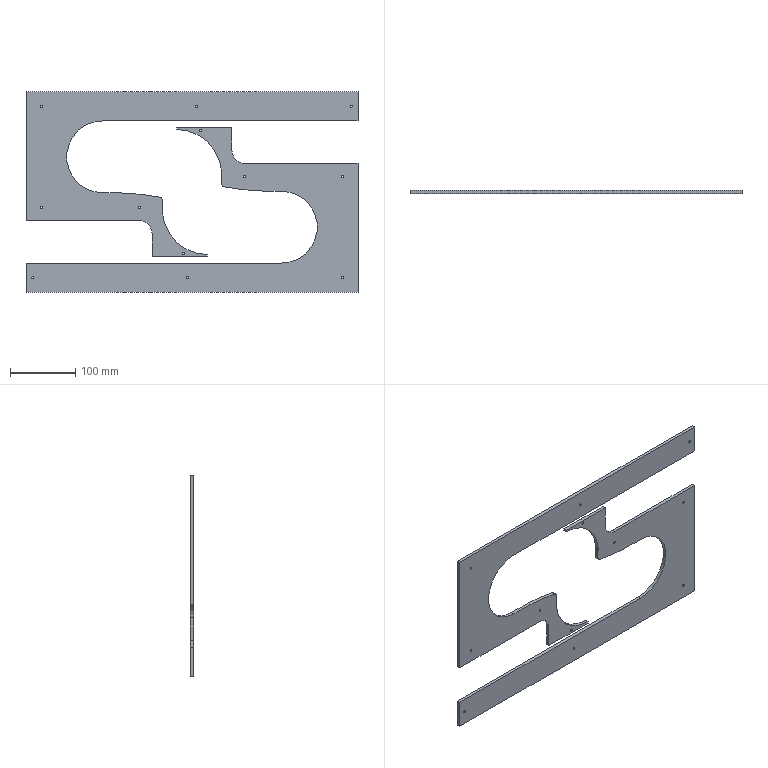CAM job | Mastercam | mm | 4 operations | part box 509.5 x 5 x 308
1. Contour (Ramp) | 3 - 3 平铣刀
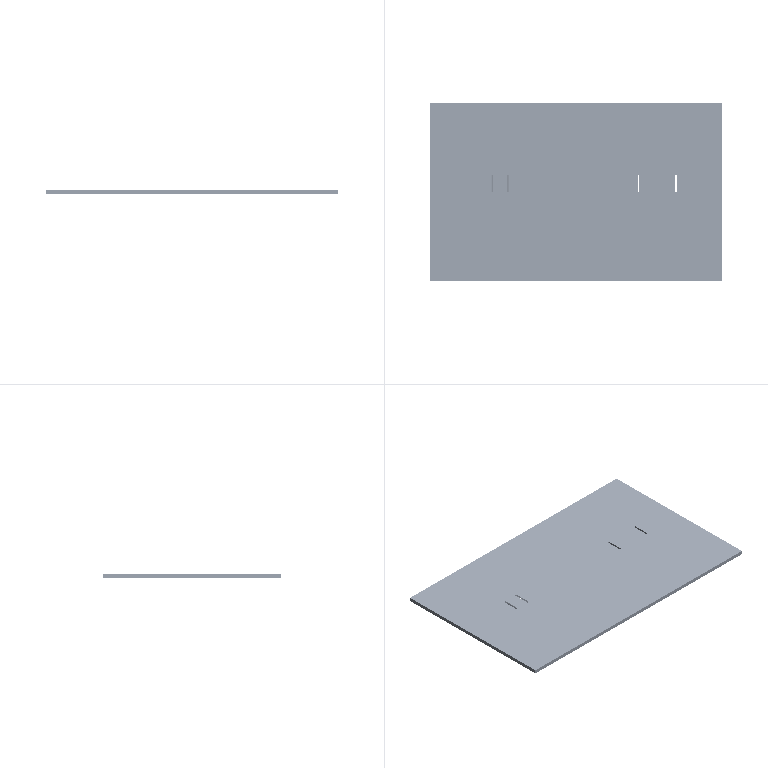2. Contour (2D) | 3 - 3 平铣刀
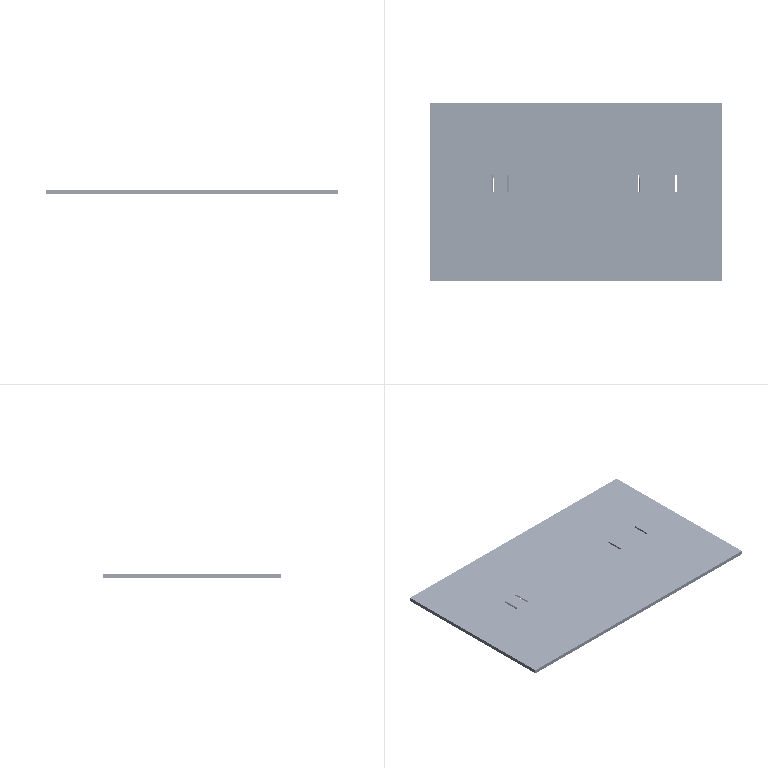3. Drill/Counterbore | 7 - 4 倒角刀
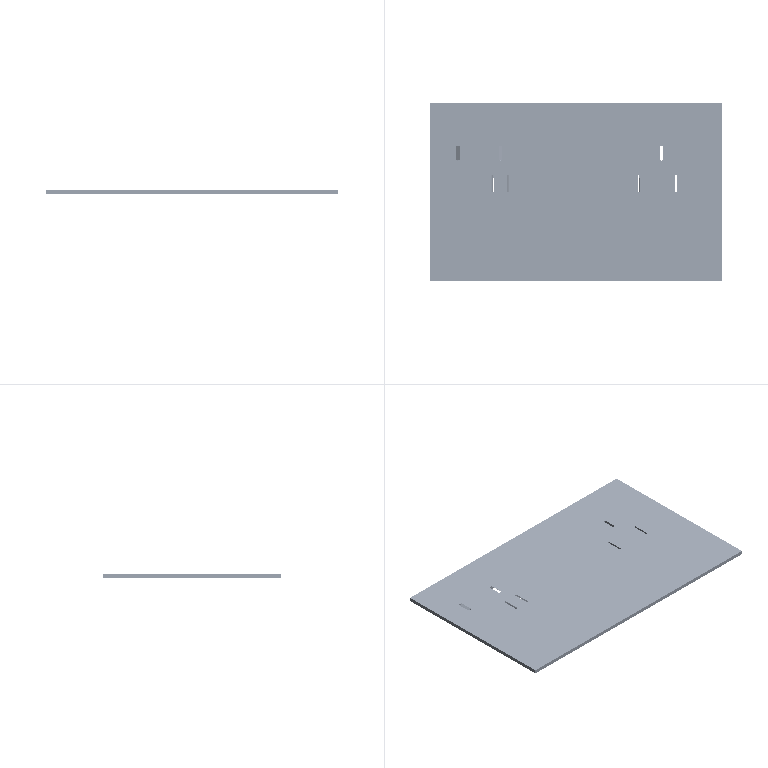4. Contour (2D chamfer) | 7 - 4 倒角刀